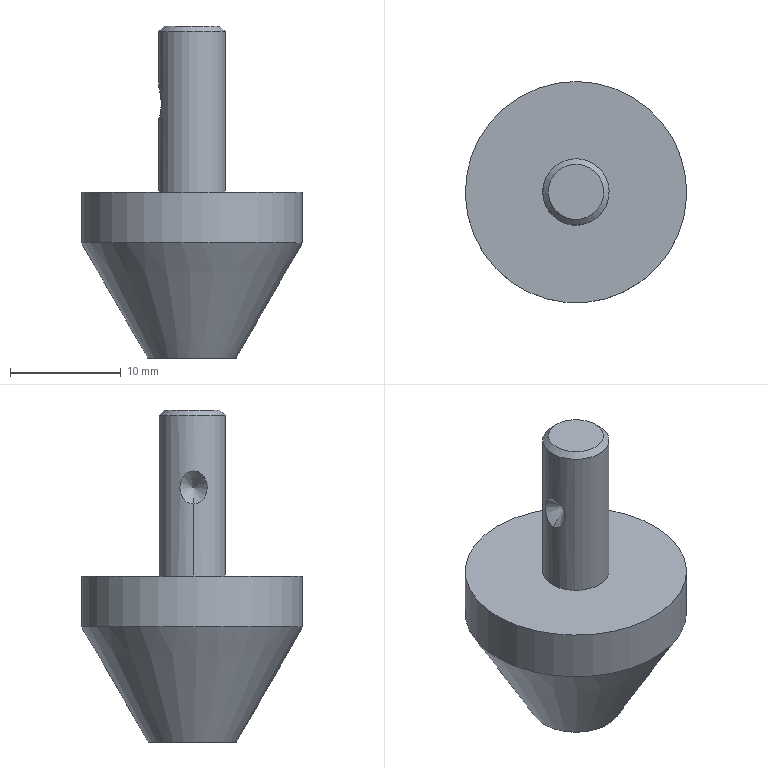Component | NX | MOLD | 1 solid | 8 faces | volume 3564 mm3 | plane 3 | cone 3 | cylinder 2 | commonest cylinder face diameters 6 x1 20 x1